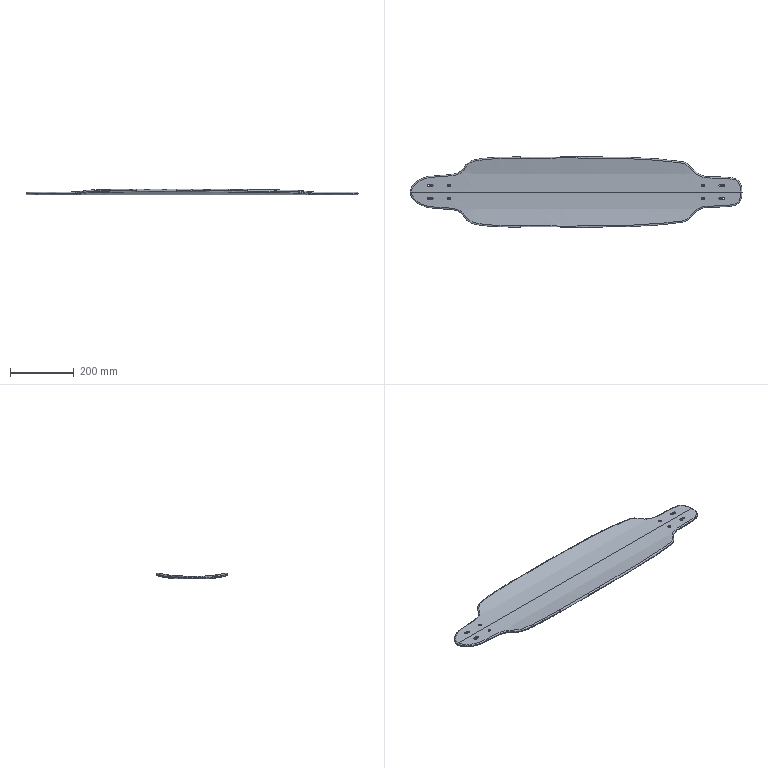Component | NX | BOARD1 | 1 solid | 62 faces | volume 1536102 mm3 | spline 20 | cylinder 16 | other 12 | cone 12 | plane 2 | commonest cylinder face diameters 5 x12 7 x4